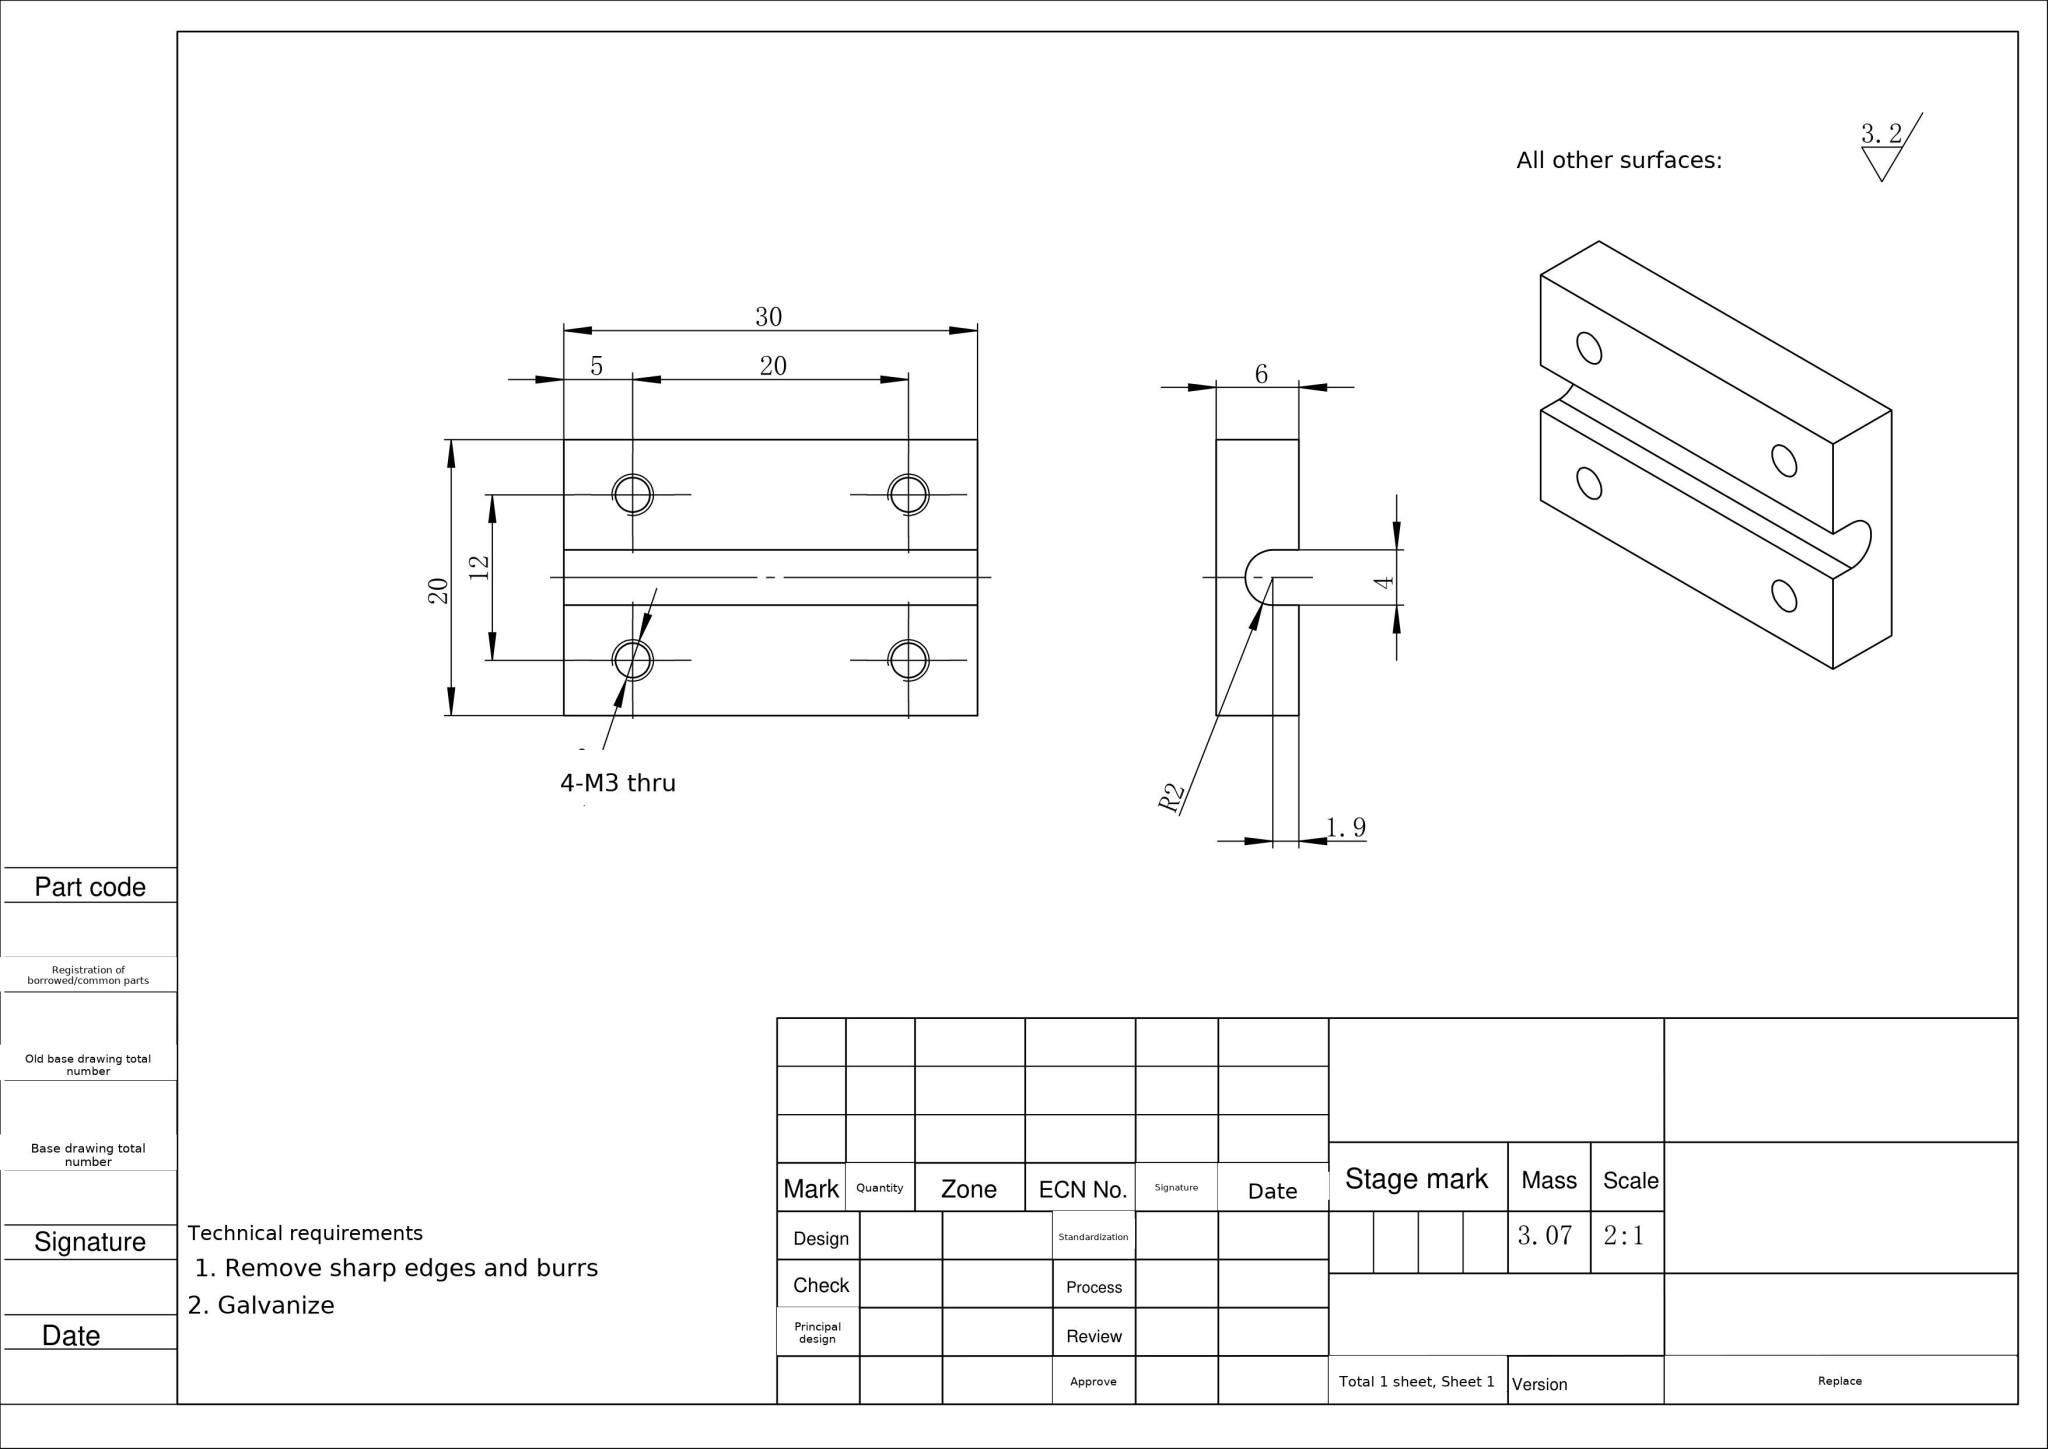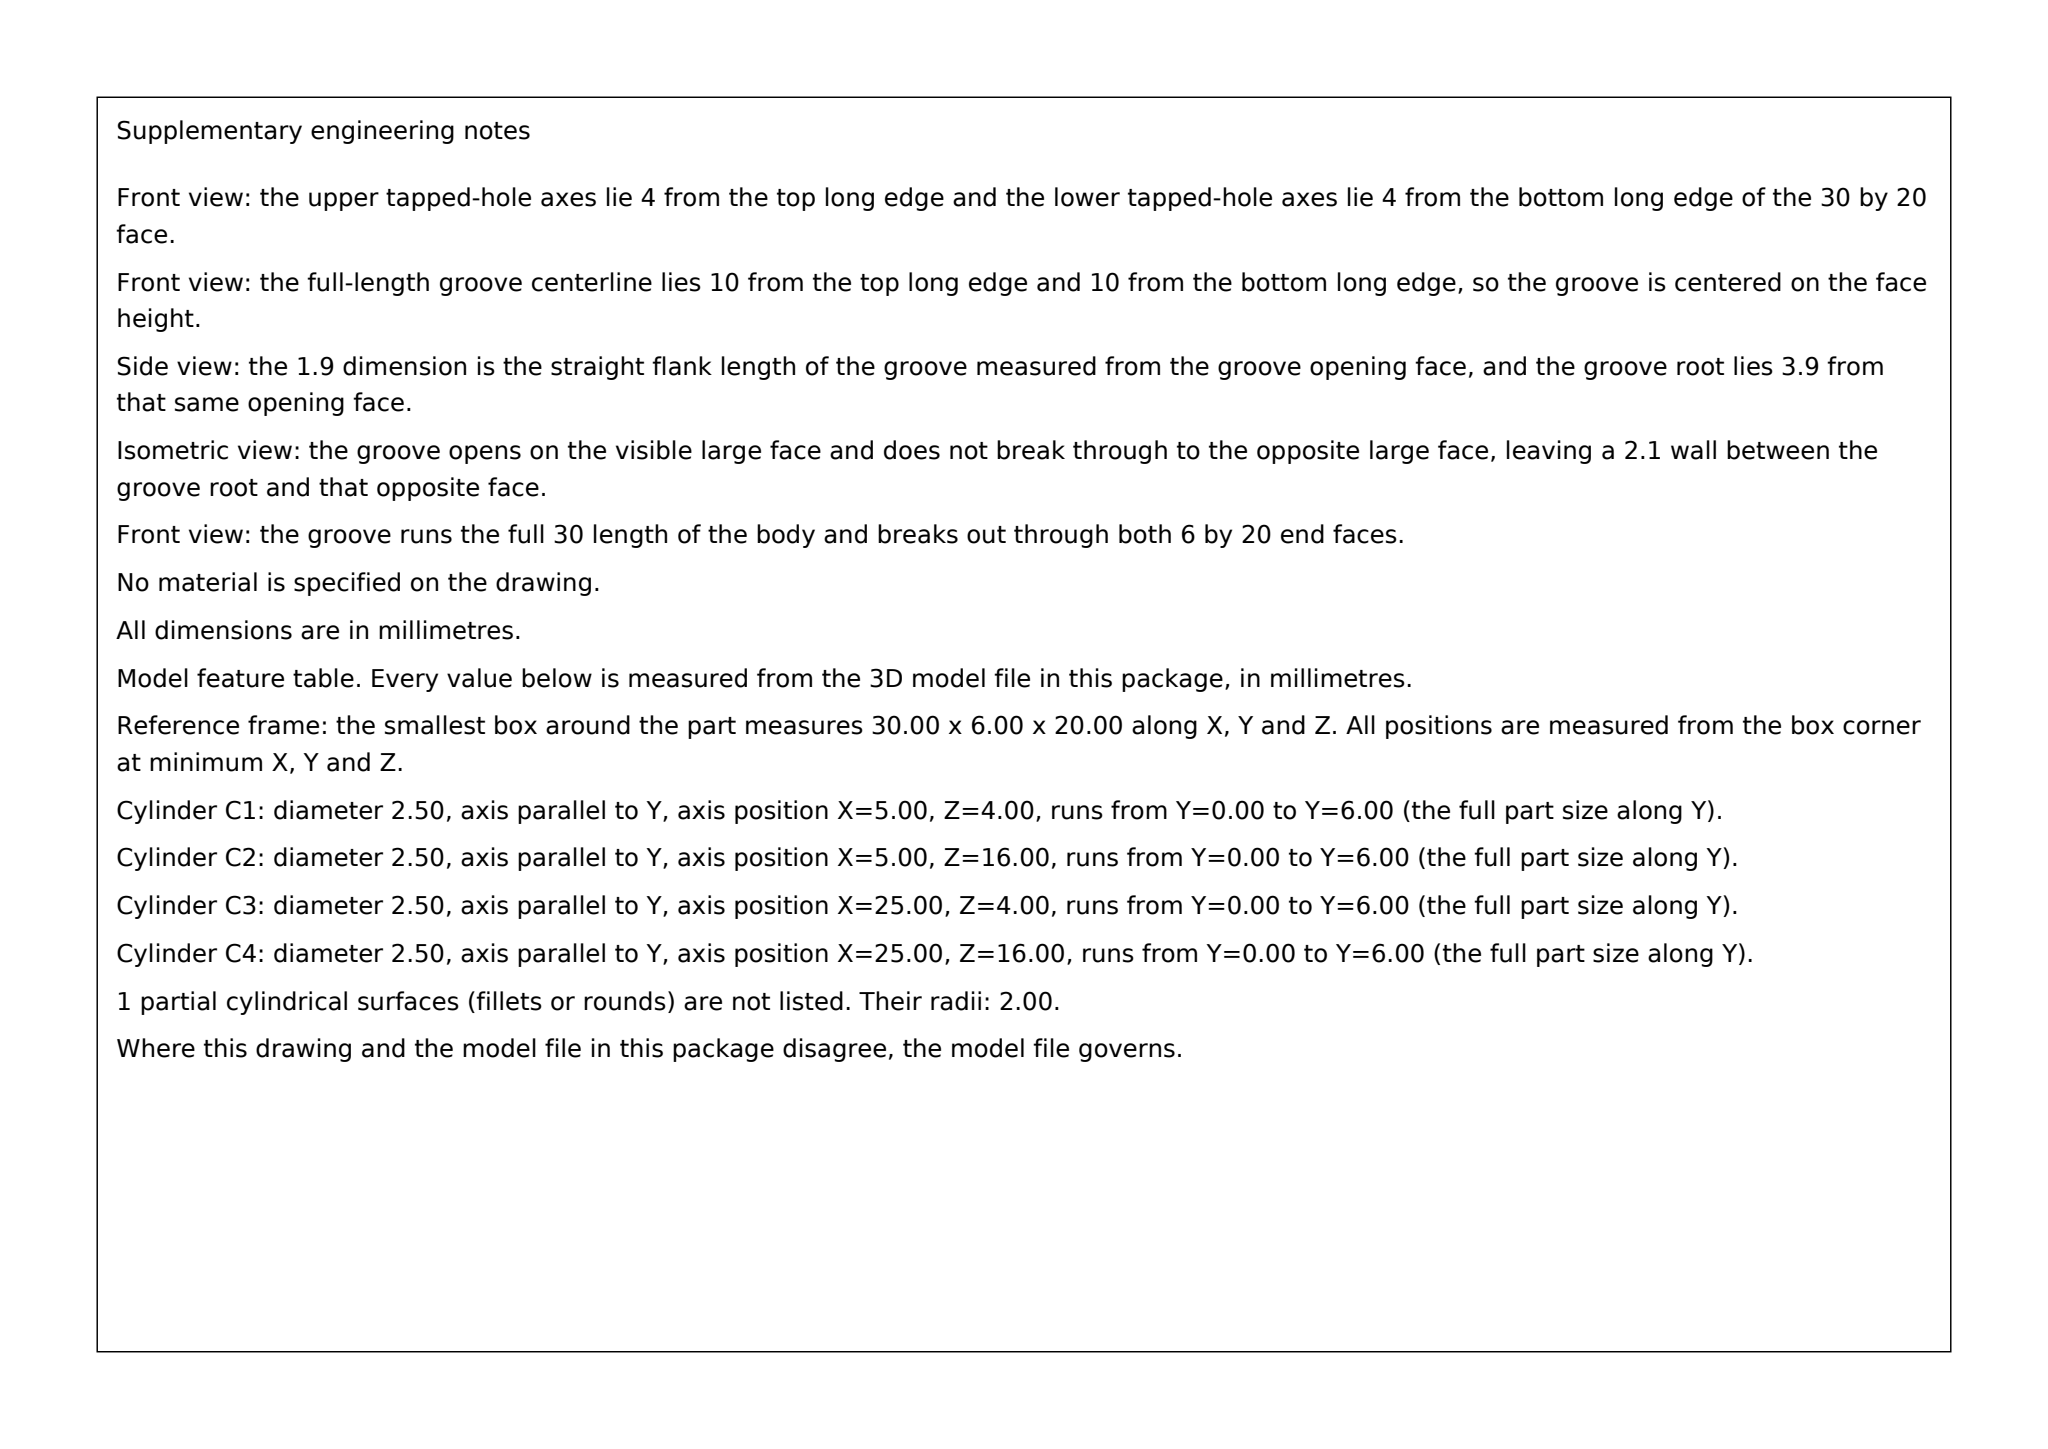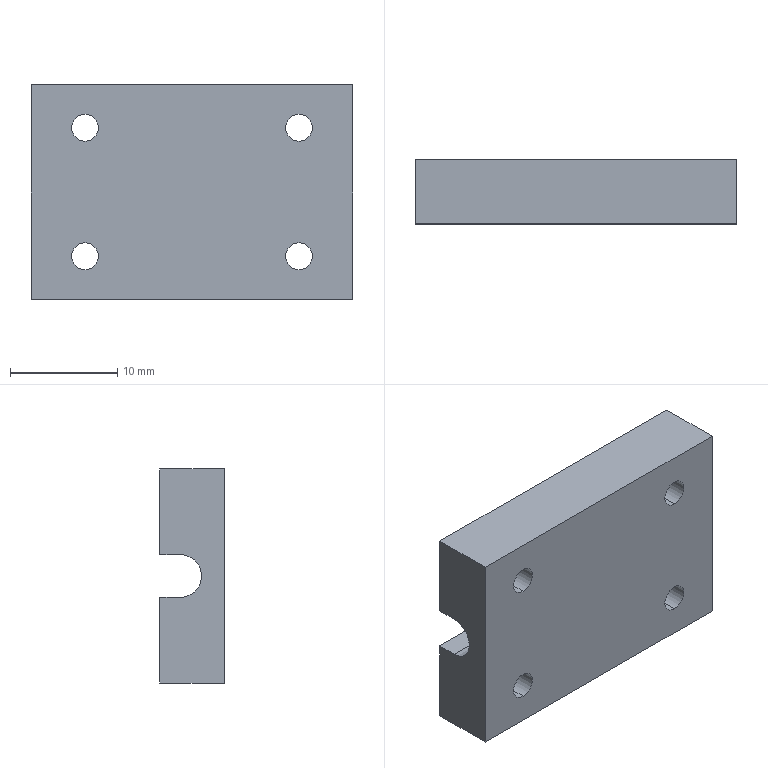Part | SolidWorks | mm | 1 solid | 18 faces | box 30 x 6 x 20 mm | volume 3066 mm3 | cylinder 9 | plane 9 | commonest cylinder face diameters 2.5 x8 4 x1
Drawing notes:
All dimensions in millimetres (mm) unless otherwise stated. | from the solid: STEP model units: mm (bbox_xyz given in mm)
GROOVE: FULL-RADIUS R2 (Ø4) THRU, 30 LONG PARALLEL TO 30 EDGE; AXIS 10 FROM BOTTOM FACE AND 1.9 FROM 6-WIDE FRONT FACE | from the solid: cylinder [4.0,"x",[null,4.1,10.0],30.0] with bbox_xyz [30,6,20] (axis 10 from z=0 face, 4.1 from y=6 face = 1.9 from y=0 face)
build123d program:
from build123d import *

# Parameters (mm, degrees)
SKETCH1_W           = 30
SKETCH1_H           = 20
BOSS_EXTRUDE2_DEPTH = 6
CUT_EXTRUDE1_DEPTH  = 170.118
M3_TAPPED_HOLE1_D   = 2.5


with BuildPart() as part:
    # Sketch1 → Boss-Extrude2 (new body)
    with BuildSketch(Plane(origin=(0, 151, -156), x_dir=(1, 0, 0), z_dir=(0, -1, 0))):
        with Locations((-165.688, 216)):
            Rectangle(SKETCH1_W, SKETCH1_H)
    extrude(amount=BOSS_EXTRUDE2_DEPTH)

    # Sketch2 → Cut-Extrude1 (cut, through all)
    with BuildSketch(Plane.ZY.offset(180.688)):
        with BuildLine():
            Line((58, 149.1), (58, 151))
            Line((58, 151), (62, 151))
            Line((62, 151), (62, 149.1))
            ThreePointArc((62, 149.1), (60, 147.1), (58, 149.1))
        make_face()
    extrude(amount=-CUT_EXTRUDE1_DEPTH, mode=Mode.SUBTRACT)

    # M3 Tapped Hole1 (through all)
    with Locations(Plane(origin=(0, 145, 0), x_dir=(-1, 0, 0), z_dir=(0, -1, 0))):
        with Locations((155.688, -66), (155.688, -54), (175.688, -66), (175.688, -54)):
            Hole(M3_TAPPED_HOLE1_D / 2)


solid = part.part
STEP:
#1=CARTESIAN_POINT('',(-155.688,151.,67.25));
#2=VERTEX_POINT('',#1);
#3=CARTESIAN_POINT('',(-155.688,151.,64.75));
#4=VERTEX_POINT('',#3);
#5=CARTESIAN_POINT('',(-155.688,151.,66.));
#6=DIRECTION('',(0.,-1.,0.));
#7=DIRECTION('',(0.,0.,-1.));
#8=AXIS2_PLACEMENT_3D('',#5,#6,#7);
#9=CIRCLE('',#8,1.25);
#10=EDGE_CURVE('',#2,#4,#9,.T.);
#11=ORIENTED_EDGE('',*,*,#10,.F.);
#12=CARTESIAN_POINT('',(-155.688,145.,67.25));
#13=VERTEX_POINT('',#12);
#14=CARTESIAN_POINT('',(-155.688,145.,67.25));
#15=DIRECTION('',(0.,-1.,0.));
#16=VECTOR('',#15,1000.);
#17=LINE('',#14,#16);
#18=EDGE_CURVE('',#2,#13,#17,.T.);
#19=ORIENTED_EDGE('',*,*,#18,.T.);
#20=CARTESIAN_POINT('',(-155.688,145.,64.75));
#21=VERTEX_POINT('',#20);
#22=CARTESIAN_POINT('',(-155.688,145.,66.));
#23=DIRECTION('',(0.,-1.,0.));
#24=DIRECTION('',(0.,0.,-1.));
#25=AXIS2_PLACEMENT_3D('',#22,#23,#24);
#26=CIRCLE('',#25,1.25);
#27=EDGE_CURVE('',#13,#21,#26,.T.);
#28=ORIENTED_EDGE('',*,*,#27,.T.);
#29=CARTESIAN_POINT('',(-155.688,145.,64.75));
#30=DIRECTION('',(0.,-1.,0.));
#31=VECTOR('',#30,1000.);
#32=LINE('',#29,#31);
#33=EDGE_CURVE('',#4,#21,#32,.T.);
#34=ORIENTED_EDGE('',*,*,#33,.F.);
#35=EDGE_LOOP('',(#11,#19,#28,#34));
#36=FACE_OUTER_BOUND('',#35,.T.);
#37=CARTESIAN_POINT('',(-155.688,145.,66.));
#38=DIRECTION('',(0.,-1.,0.));
#39=DIRECTION('',(0.,0.,-1.));
#40=AXIS2_PLACEMENT_3D('',#37,#38,#39);
#41=CYLINDRICAL_SURFACE('',#40,1.25);
#42=ADVANCED_FACE('',(#36),#41,.F.);
#43=CARTESIAN_POINT('',(-155.688,151.,55.25));
#44=VERTEX_POINT('',#43);
#45=CARTESIAN_POINT('',(-155.688,151.,52.75));
#46=VERTEX_POINT('',#45);
#47=CARTESIAN_POINT('',(-155.688,151.,54.));
#48=DIRECTION('',(0.,-1.,0.));
#49=DIRECTION('',(0.,0.,-1.));
#50=AXIS2_PLACEMENT_3D('',#47,#48,#49);
#51=CIRCLE('',#50,1.25);
#52=EDGE_CURVE('',#44,#46,#51,.T.);
#53=ORIENTED_EDGE('',*,*,#52,.F.);
#54=CARTESIAN_POINT('',(-155.688,145.,55.25));
#55=VERTEX_POINT('',#54);
#56=CARTESIAN_POINT('',(-155.688,145.,55.25));
#57=DIRECTION('',(0.,-1.,0.));
#58=VECTOR('',#57,1000.);
#59=LINE('',#56,#58);
#60=EDGE_CURVE('',#44,#55,#59,.T.);
#61=ORIENTED_EDGE('',*,*,#60,.T.);
#62=CARTESIAN_POINT('',(-155.688,145.,52.75));
#63=VERTEX_POINT('',#62);
#64=CARTESIAN_POINT('',(-155.688,145.,54.));
#65=DIRECTION('',(0.,-1.,0.));
#66=DIRECTION('',(0.,0.,-1.));
#67=AXIS2_PLACEMENT_3D('',#64,#65,#66);
#68=CIRCLE('',#67,1.25);
#69=EDGE_CURVE('',#55,#63,#68,.T.);
#70=ORIENTED_EDGE('',*,*,#69,.T.);
#71=CARTESIAN_POINT('',(-155.688,145.,52.75));
#72=DIRECTION('',(0.,-1.,0.));
#73=VECTOR('',#72,1000.);
#74=LINE('',#71,#73);
#75=EDGE_CURVE('',#46,#63,#74,.T.);
#76=ORIENTED_EDGE('',*,*,#75,.F.);
#77=EDGE_LOOP('',(#53,#61,#70,#76));
#78=FACE_OUTER_BOUND('',#77,.T.);
#79=CARTESIAN_POINT('',(-155.688,145.,54.));
#80=DIRECTION('',(0.,-1.,0.));
#81=DIRECTION('',(0.,0.,-1.));
#82=AXIS2_PLACEMENT_3D('',#79,#80,#81);
#83=CYLINDRICAL_SURFACE('',#82,1.25);
#84=ADVANCED_FACE('',(#78),#83,.F.);
#85=CARTESIAN_POINT('',(-175.688,151.,67.25));
#86=VERTEX_POINT('',#85);
#87=CARTESIAN_POINT('',(-175.688,151.,64.75));
#88=VERTEX_POINT('',#87);
#89=CARTESIAN_POINT('',(-175.688,151.,66.));
#90=DIRECTION('',(0.,-1.,0.));
#91=DIRECTION('',(0.,0.,-1.));
#92=AXIS2_PLACEMENT_3D('',#89,#90,#91);
#93=CIRCLE('',#92,1.25);
#94=EDGE_CURVE('',#86,#88,#93,.T.);
#95=ORIENTED_EDGE('',*,*,#94,.F.);
#96=CARTESIAN_POINT('',(-175.688,145.,67.25));
#97=VERTEX_POINT('',#96);
#98=CARTESIAN_POINT('',(-175.688,145.,67.25));
#99=DIRECTION('',(0.,-1.,0.));
#100=VECTOR('',#99,1000.);
#101=LINE('',#98,#100);
#102=EDGE_CURVE('',#86,#97,#101,.T.);
#103=ORIENTED_EDGE('',*,*,#102,.T.);
#104=CARTESIAN_POINT('',(-175.688,145.,64.75));
#105=VERTEX_POINT('',#104);
#106=CARTESIAN_POINT('',(-175.688,145.,66.));
#107=DIRECTION('',(0.,-1.,0.));
#108=DIRECTION('',(0.,0.,-1.));
#109=AXIS2_PLACEMENT_3D('',#106,#107,#108);
#110=CIRCLE('',#109,1.25);
#111=EDGE_CURVE('',#97,#105,#110,.T.);
#112=ORIENTED_EDGE('',*,*,#111,.T.);
#113=CARTESIAN_POINT('',(-175.688,145.,64.75));
#114=DIRECTION('',(0.,-1.,0.));
#115=VECTOR('',#114,1000.);
#116=LINE('',#113,#115);
#117=EDGE_CURVE('',#88,#105,#116,.T.);
#118=ORIENTED_EDGE('',*,*,#117,.F.);
#119=EDGE_LOOP('',(#95,#103,#112,#118));
#120=FACE_OUTER_BOUND('',#119,.T.);
#121=CARTESIAN_POINT('',(-175.688,145.,66.));
#122=DIRECTION('',(0.,-1.,0.));
#123=DIRECTION('',(0.,0.,-1.));
#124=AXIS2_PLACEMENT_3D('',#121,#122,#123);
#125=CYLINDRICAL_SURFACE('',#124,1.25);
#126=ADVANCED_FACE('',(#120),#125,.F.);
#127=CARTESIAN_POINT('',(-175.688,151.,55.25));
#128=VERTEX_POINT('',#127);
#129=CARTESIAN_POINT('',(-175.688,151.,52.75));
#130=VERTEX_POINT('',#129);
#131=CARTESIAN_POINT('',(-175.688,151.,54.));
#132=DIRECTION('',(0.,-1.,0.));
#133=DIRECTION('',(0.,0.,-1.));
#134=AXIS2_PLACEMENT_3D('',#131,#132,#133);
#135=CIRCLE('',#134,1.25);
#136=EDGE_CURVE('',#128,#130,#135,.T.);
#137=ORIENTED_EDGE('',*,*,#136,.F.);
#138=CARTESIAN_POINT('',(-175.688,145.,55.25));
#139=VERTEX_POINT('',#138);
#140=CARTESIAN_POINT('',(-175.688,145.,55.25));
#141=DIRECTION('',(0.,-1.,0.));
#142=VECTOR('',#141,1000.);
#143=LINE('',#140,#142);
#144=EDGE_CURVE('',#128,#139,#143,.T.);
#145=ORIENTED_EDGE('',*,*,#144,.T.);
#146=CARTESIAN_POINT('',(-175.688,145.,52.75));
#147=VERTEX_POINT('',#146);
#148=CARTESIAN_POINT('',(-175.688,145.,54.));
#149=DIRECTION('',(0.,-1.,0.));
#150=DIRECTION('',(0.,0.,-1.));
#151=AXIS2_PLACEMENT_3D('',#148,#149,#150);
#152=CIRCLE('',#151,1.25);
#153=EDGE_CURVE('',#139,#147,#152,.T.);
#154=ORIENTED_EDGE('',*,*,#153,.T.);
#155=CARTESIAN_POINT('',(-175.688,145.,52.75));
#156=DIRECTION('',(0.,-1.,0.));
#157=VECTOR('',#156,1000.);
#158=LINE('',#155,#157);
#159=EDGE_CURVE('',#130,#147,#158,.T.);
#160=ORIENTED_EDGE('',*,*,#159,.F.);
#161=EDGE_LOOP('',(#137,#145,#154,#160));
#162=FACE_OUTER_BOUND('',#161,.T.);
#163=CARTESIAN_POINT('',(-175.688,145.,54.));
#164=DIRECTION('',(0.,-1.,0.));
#165=DIRECTION('',(0.,0.,-1.));
#166=AXIS2_PLACEMENT_3D('',#163,#164,#165);
#167=CYLINDRICAL_SURFACE('',#166,1.25);
#168=ADVANCED_FACE('',(#162),#167,.F.);
#169=CARTESIAN_POINT('',(-155.688,151.,54.));
#170=DIRECTION('',(0.,-1.,0.));
#171=DIRECTION('',(0.,0.,-1.));
#172=AXIS2_PLACEMENT_3D('',#169,#170,#171);
#173=CIRCLE('',#172,1.25);
#174=EDGE_CURVE('',#46,#44,#173,.T.);
#175=ORIENTED_EDGE('',*,*,#174,.T.);
#176=ORIENTED_EDGE('',*,*,#52,.T.);
#177=EDGE_LOOP('',(#175,#176));
#178=FACE_BOUND('',#177,.T.);
#179=CARTESIAN_POINT('',(-175.688,151.,54.));
#180=DIRECTION('',(0.,-1.,0.));
#181=DIRECTION('',(0.,0.,-1.));
#182=AXIS2_PLACEMENT_3D('',#179,#180,#181);
#183=CIRCLE('',#182,1.25);
#184=EDGE_CURVE('',#130,#128,#183,.T.);
#185=ORIENTED_EDGE('',*,*,#184,.T.);
#186=ORIENTED_EDGE('',*,*,#136,.T.);
#187=EDGE_LOOP('',(#185,#186));
#188=FACE_BOUND('',#187,.T.);
#189=CARTESIAN_POINT('',(-180.688,151.,58.));
#190=VERTEX_POINT('',#189);
#191=CARTESIAN_POINT('',(-180.688,151.,50.));
#192=VERTEX_POINT('',#191);
#193=CARTESIAN_POINT('',(-180.688,151.,70.));
#194=DIRECTION('',(0.,-0.,-1.));
#195=VECTOR('',#194,1000.);
#196=LINE('',#193,#195);
#197=EDGE_CURVE('',#190,#192,#196,.T.);
#198=ORIENTED_EDGE('',*,*,#197,.F.);
#199=CARTESIAN_POINT('',(-150.688,151.,58.));
#200=VERTEX_POINT('',#199);
#201=CARTESIAN_POINT('',(-150.688,151.,58.));
#202=DIRECTION('',(-1.,0.,0.));
#203=VECTOR('',#202,1000.);
#204=LINE('',#201,#203);
#205=EDGE_CURVE('',#200,#190,#204,.T.);
#206=ORIENTED_EDGE('',*,*,#205,.F.);
#207=CARTESIAN_POINT('',(-150.688,151.,50.));
#208=VERTEX_POINT('',#207);
#209=CARTESIAN_POINT('',(-150.688,151.,70.));
#210=DIRECTION('',(0.,0.,1.));
#211=VECTOR('',#210,1000.);
#212=LINE('',#209,#211);
#213=EDGE_CURVE('',#208,#200,#212,.T.);
#214=ORIENTED_EDGE('',*,*,#213,.F.);
#215=CARTESIAN_POINT('',(-180.688,151.,50.));
#216=DIRECTION('',(1.,0.,0.));
#217=VECTOR('',#216,1000.);
#218=LINE('',#215,#217);
#219=EDGE_CURVE('',#192,#208,#218,.T.);
#220=ORIENTED_EDGE('',*,*,#219,.F.);
#221=EDGE_LOOP('',(#198,#206,#214,#220));
#222=FACE_OUTER_BOUND('',#221,.T.);
#223=CARTESIAN_POINT('',(0.,151.,-0.));
#224=DIRECTION('',(0.,-1.,0.));
#225=DIRECTION('',(0.,-0.,-1.));
#226=AXIS2_PLACEMENT_3D('',#223,#224,#225);
#227=PLANE('',#226);
#228=ADVANCED_FACE('',(#178,#188,#222),#227,.F.);
#229=CARTESIAN_POINT('',(-180.688,149.1,58.));
#230=VERTEX_POINT('',#229);
#231=CARTESIAN_POINT('',(-180.688,149.1,62.));
#232=VERTEX_POINT('',#231);
#233=CARTESIAN_POINT('',(-180.688,149.1,60.));
#234=DIRECTION('',(-1.,0.,0.));
#235=DIRECTION('',(0.,0.,1.));
#236=AXIS2_PLACEMENT_3D('',#233,#234,#235);
#237=CIRCLE('',#236,2.);
#238=EDGE_CURVE('',#230,#232,#237,.T.);
#239=ORIENTED_EDGE('',*,*,#238,.F.);
#240=CARTESIAN_POINT('',(-180.688,149.1,58.));
#241=DIRECTION('',(0.,-1.,0.));
#242=VECTOR('',#241,1000.);
#243=LINE('',#240,#242);
#244=EDGE_CURVE('',#190,#230,#243,.T.);
#245=ORIENTED_EDGE('',*,*,#244,.F.);
#246=ORIENTED_EDGE('',*,*,#197,.T.);
#247=CARTESIAN_POINT('',(-180.688,145.,50.));
#248=VERTEX_POINT('',#247);
#249=CARTESIAN_POINT('',(-180.688,145.,50.));
#250=DIRECTION('',(0.,1.,-0.));
#251=VECTOR('',#250,1000.);
#252=LINE('',#249,#251);
#253=EDGE_CURVE('',#248,#192,#252,.T.);
#254=ORIENTED_EDGE('',*,*,#253,.F.);
#255=CARTESIAN_POINT('',(-180.688,145.,70.));
#256=VERTEX_POINT('',#255);
#257=CARTESIAN_POINT('',(-180.688,145.,70.));
#258=DIRECTION('',(0.,-0.,-1.));
#259=VECTOR('',#258,1000.);
#260=LINE('',#257,#259);
#261=EDGE_CURVE('',#256,#248,#260,.T.);
#262=ORIENTED_EDGE('',*,*,#261,.F.);
#263=CARTESIAN_POINT('',(-180.688,151.,70.));
#264=VERTEX_POINT('',#263);
#265=CARTESIAN_POINT('',(-180.688,145.,70.));
#266=DIRECTION('',(0.,1.,-0.));
#267=VECTOR('',#266,1000.);
#268=LINE('',#265,#267);
#269=EDGE_CURVE('',#256,#264,#268,.T.);
#270=ORIENTED_EDGE('',*,*,#269,.T.);
#271=CARTESIAN_POINT('',(-180.688,151.,62.));
#272=VERTEX_POINT('',#271);
#273=CARTESIAN_POINT('',(-180.688,151.,70.));
#274=DIRECTION('',(0.,-0.,-1.));
#275=VECTOR('',#274,1000.);
#276=LINE('',#273,#275);
#277=EDGE_CURVE('',#264,#272,#276,.T.);
#278=ORIENTED_EDGE('',*,*,#277,.T.);
#279=CARTESIAN_POINT('',(-180.688,151.,62.));
#280=DIRECTION('',(0.,1.,0.));
#281=VECTOR('',#280,1000.);
#282=LINE('',#279,#281);
#283=EDGE_CURVE('',#232,#272,#282,.T.);
#284=ORIENTED_EDGE('',*,*,#283,.F.);
#285=EDGE_LOOP('',(#239,#245,#246,#254,#262,#270,#278,#284));
#286=FACE_OUTER_BOUND('',#285,.T.);
#287=CARTESIAN_POINT('',(-180.688,145.,70.));
#288=DIRECTION('',(1.,0.,0.));
#289=DIRECTION('',(0.,0.,-1.));
#290=AXIS2_PLACEMENT_3D('',#287,#288,#289);
#291=PLANE('',#290);
#292=ADVANCED_FACE('',(#286),#291,.F.);
#293=ORIENTED_EDGE('',*,*,#219,.T.);
#294=CARTESIAN_POINT('',(-150.688,145.,50.));
#295=VERTEX_POINT('',#294);
#296=CARTESIAN_POINT('',(-150.688,145.,50.));
#297=DIRECTION('',(0.,1.,-0.));
#298=VECTOR('',#297,1000.);
#299=LINE('',#296,#298);
#300=EDGE_CURVE('',#295,#208,#299,.T.);
#301=ORIENTED_EDGE('',*,*,#300,.F.);
#302=CARTESIAN_POINT('',(-180.688,145.,50.));
#303=DIRECTION('',(1.,0.,0.));
#304=VECTOR('',#303,1000.);
#305=LINE('',#302,#304);
#306=EDGE_CURVE('',#248,#295,#305,.T.);
#307=ORIENTED_EDGE('',*,*,#306,.F.);
#308=ORIENTED_EDGE('',*,*,#253,.T.);
#309=EDGE_LOOP('',(#293,#301,#307,#308));
#310=FACE_OUTER_BOUND('',#309,.T.);
#311=CARTESIAN_POINT('',(-180.688,145.,50.));
#312=DIRECTION('',(0.,0.,1.));
#313=DIRECTION('',(0.,-1.,0.));
#314=AXIS2_PLACEMENT_3D('',#311,#312,#313);
#315=PLANE('',#314);
#316=ADVANCED_FACE('',(#310),#315,.F.);
#317=ORIENTED_EDGE('',*,*,#213,.T.);
#318=CARTESIAN_POINT('',(-150.688,149.1,58.));
#319=VERTEX_POINT('',#318);
#320=CARTESIAN_POINT('',(-150.688,149.1,58.));
#321=DIRECTION('',(0.,-1.,0.));
#322=VECTOR('',#321,1000.);
#323=LINE('',#320,#322);
#324=EDGE_CURVE('',#200,#319,#323,.T.);
#325=ORIENTED_EDGE('',*,*,#324,.T.);
#326=CARTESIAN_POINT('',(-150.688,149.1,62.));
#327=VERTEX_POINT('',#326);
#328=CARTESIAN_POINT('',(-150.688,149.1,60.));
#329=DIRECTION('',(-1.,0.,0.));
#330=DIRECTION('',(0.,0.,1.));
#331=AXIS2_PLACEMENT_3D('',#328,#329,#330);
#332=CIRCLE('',#331,2.);
#333=EDGE_CURVE('',#319,#327,#332,.T.);
#334=ORIENTED_EDGE('',*,*,#333,.T.);
#335=CARTESIAN_POINT('',(-150.688,151.,62.));
#336=VERTEX_POINT('',#335);
#337=CARTESIAN_POINT('',(-150.688,151.,62.));
#338=DIRECTION('',(0.,1.,0.));
#339=VECTOR('',#338,1000.);
#340=LINE('',#337,#339);
#341=EDGE_CURVE('',#327,#336,#340,.T.);
#342=ORIENTED_EDGE('',*,*,#341,.T.);
#343=CARTESIAN_POINT('',(-150.688,151.,70.));
#344=VERTEX_POINT('',#343);
#345=CARTESIAN_POINT('',(-150.688,151.,70.));
#346=DIRECTION('',(0.,0.,1.));
#347=VECTOR('',#346,1000.);
#348=LINE('',#345,#347);
#349=EDGE_CURVE('',#336,#344,#348,.T.);
#350=ORIENTED_EDGE('',*,*,#349,.T.);
#351=CARTESIAN_POINT('',(-150.688,145.,70.));
#352=VERTEX_POINT('',#351);
#353=CARTESIAN_POINT('',(-150.688,145.,70.));
#354=DIRECTION('',(0.,1.,-0.));
#355=VECTOR('',#354,1000.);
#356=LINE('',#353,#355);
#357=EDGE_CURVE('',#352,#344,#356,.T.);
#358=ORIENTED_EDGE('',*,*,#357,.F.);
#359=CARTESIAN_POINT('',(-150.688,145.,70.));
#360=DIRECTION('',(0.,0.,1.));
#361=VECTOR('',#360,1000.);
#362=LINE('',#359,#361);
#363=EDGE_CURVE('',#295,#352,#362,.T.);
#364=ORIENTED_EDGE('',*,*,#363,.F.);
#365=ORIENTED_EDGE('',*,*,#300,.T.);
#366=EDGE_LOOP('',(#317,#325,#334,#342,#350,#358,#364,#365));
#367=FACE_OUTER_BOUND('',#366,.T.);
#368=CARTESIAN_POINT('',(-150.688,145.,70.));
#369=DIRECTION('',(-1.,0.,0.));
#370=DIRECTION('',(0.,0.,1.));
#371=AXIS2_PLACEMENT_3D('',#368,#369,#370);
#372=PLANE('',#371);
#373=ADVANCED_FACE('',(#367),#372,.F.);
#374=CARTESIAN_POINT('',(-180.688,151.,70.));
#375=DIRECTION('',(-1.,0.,0.));
#376=VECTOR('',#375,1000.);
#377=LINE('',#374,#376);
#378=EDGE_CURVE('',#344,#264,#377,.T.);
#379=ORIENTED_EDGE('',*,*,#378,.T.);
#380=ORIENTED_EDGE('',*,*,#269,.F.);
#381=CARTESIAN_POINT('',(-180.688,145.,70.));
#382=DIRECTION('',(-1.,0.,0.));
#383=VECTOR('',#382,1000.);
#384=LINE('',#381,#383);
#385=EDGE_CURVE('',#352,#256,#384,.T.);
#386=ORIENTED_EDGE('',*,*,#385,.F.);
#387=ORIENTED_EDGE('',*,*,#357,.T.);
#388=EDGE_LOOP('',(#379,#380,#386,#387));
#389=FACE_OUTER_BOUND('',#388,.T.);
#390=CARTESIAN_POINT('',(-180.688,145.,70.));
#391=DIRECTION('',(0.,-0.,-1.));
#392=DIRECTION('',(0.,1.,-0.));
#393=AXIS2_PLACEMENT_3D('',#390,#391,#392);
#394=PLANE('',#393);
#395=ADVANCED_FACE('',(#389),#394,.F.);
#396=CARTESIAN_POINT('',(-155.688,145.,66.));
#397=DIRECTION('',(0.,-1.,0.));
#398=DIRECTION('',(0.,0.,-1.));
#399=AXIS2_PLACEMENT_3D('',#396,#397,#398);
#400=CIRCLE('',#399,1.25);
#401=EDGE_CURVE('',#21,#13,#400,.T.);
#402=ORIENTED_EDGE('',*,*,#401,.F.);
#403=ORIENTED_EDGE('',*,*,#27,.F.);
#404=EDGE_LOOP('',(#402,#403));
#405=FACE_BOUND('',#404,.T.);
#406=CARTESIAN_POINT('',(-155.688,145.,54.));
#407=DIRECTION('',(0.,-1.,0.));
#408=DIRECTION('',(0.,0.,-1.));
#409=AXIS2_PLACEMENT_3D('',#406,#407,#408);
#410=CIRCLE('',#409,1.25);
#411=EDGE_CURVE('',#63,#55,#410,.T.);
#412=ORIENTED_EDGE('',*,*,#411,.F.);
#413=ORIENTED_EDGE('',*,*,#69,.F.);
#414=EDGE_LOOP('',(#412,#413));
#415=FACE_BOUND('',#414,.T.);
#416=CARTESIAN_POINT('',(-175.688,145.,66.));
#417=DIRECTION('',(0.,-1.,0.));
#418=DIRECTION('',(0.,0.,-1.));
#419=AXIS2_PLACEMENT_3D('',#416,#417,#418);
#420=CIRCLE('',#419,1.25);
#421=EDGE_CURVE('',#105,#97,#420,.T.);
#422=ORIENTED_EDGE('',*,*,#421,.F.);
#423=ORIENTED_EDGE('',*,*,#111,.F.);
#424=EDGE_LOOP('',(#422,#423));
#425=FACE_BOUND('',#424,.T.);
#426=CARTESIAN_POINT('',(-175.688,145.,54.));
#427=DIRECTION('',(0.,-1.,0.));
#428=DIRECTION('',(0.,0.,-1.));
#429=AXIS2_PLACEMENT_3D('',#426,#427,#428);
#430=CIRCLE('',#429,1.25);
#431=EDGE_CURVE('',#147,#139,#430,.T.);
#432=ORIENTED_EDGE('',*,*,#431,.F.);
#433=ORIENTED_EDGE('',*,*,#153,.F.);
#434=EDGE_LOOP('',(#432,#433));
#435=FACE_BOUND('',#434,.T.);
#436=ORIENTED_EDGE('',*,*,#261,.T.);
#437=ORIENTED_EDGE('',*,*,#306,.T.);
#438=ORIENTED_EDGE('',*,*,#363,.T.);
#439=ORIENTED_EDGE('',*,*,#385,.T.);
#440=EDGE_LOOP('',(#436,#437,#438,#439));
#441=FACE_OUTER_BOUND('',#440,.T.);
#442=CARTESIAN_POINT('',(0.,145.,-0.));
#443=DIRECTION('',(0.,-1.,0.));
#444=DIRECTION('',(0.,-0.,-1.));
#445=AXIS2_PLACEMENT_3D('',#442,#443,#444);
#446=PLANE('',#445);
#447=ADVANCED_FACE('',(#405,#415,#425,#435,#441),#446,.T.);
#448=CARTESIAN_POINT('',(-155.688,151.,66.));
#449=DIRECTION('',(0.,-1.,0.));
#450=DIRECTION('',(0.,0.,-1.));
#451=AXIS2_PLACEMENT_3D('',#448,#449,#450);
#452=CIRCLE('',#451,1.25);
#453=EDGE_CURVE('',#4,#2,#452,.T.);
#454=ORIENTED_EDGE('',*,*,#453,.T.);
#455=ORIENTED_EDGE('',*,*,#10,.T.);
#456=EDGE_LOOP('',(#454,#455));
#457=FACE_BOUND('',#456,.T.);
#458=CARTESIAN_POINT('',(-175.688,151.,66.));
#459=DIRECTION('',(0.,-1.,0.));
#460=DIRECTION('',(0.,0.,-1.));
#461=AXIS2_PLACEMENT_3D('',#458,#459,#460);
#462=CIRCLE('',#461,1.25);
#463=EDGE_CURVE('',#88,#86,#462,.T.);
#464=ORIENTED_EDGE('',*,*,#463,.T.);
#465=ORIENTED_EDGE('',*,*,#94,.T.);
#466=EDGE_LOOP('',(#464,#465));
#467=FACE_BOUND('',#466,.T.);
#468=ORIENTED_EDGE('',*,*,#349,.F.);
#469=CARTESIAN_POINT('',(-150.688,151.,62.));
#470=DIRECTION('',(-1.,0.,0.));
#471=VECTOR('',#470,1000.);
#472=LINE('',#469,#471);
#473=EDGE_CURVE('',#336,#272,#472,.T.);
#474=ORIENTED_EDGE('',*,*,#473,.T.);
#475=ORIENTED_EDGE('',*,*,#277,.F.);
#476=ORIENTED_EDGE('',*,*,#378,.F.);
#477=EDGE_LOOP('',(#468,#474,#475,#476));
#478=FACE_OUTER_BOUND('',#477,.T.);
#479=CARTESIAN_POINT('',(0.,151.,-0.));
#480=DIRECTION('',(0.,-1.,0.));
#481=DIRECTION('',(0.,-0.,-1.));
#482=AXIS2_PLACEMENT_3D('',#479,#480,#481);
#483=PLANE('',#482);
#484=ADVANCED_FACE('',(#457,#467,#478),#483,.F.);
#485=ORIENTED_EDGE('',*,*,#238,.T.);
#486=CARTESIAN_POINT('',(-150.688,149.1,62.));
#487=DIRECTION('',(-1.,0.,0.));
#488=VECTOR('',#487,1000.);
#489=LINE('',#486,#488);
#490=EDGE_CURVE('',#327,#232,#489,.T.);
#491=ORIENTED_EDGE('',*,*,#490,.F.);
#492=ORIENTED_EDGE('',*,*,#333,.F.);
#493=CARTESIAN_POINT('',(-150.688,149.1,58.));
#494=DIRECTION('',(-1.,0.,0.));
#495=VECTOR('',#494,1000.);
#496=LINE('',#493,#495);
#497=EDGE_CURVE('',#319,#230,#496,.T.);
#498=ORIENTED_EDGE('',*,*,#497,.T.);
#499=EDGE_LOOP('',(#485,#491,#492,#498));
#500=FACE_OUTER_BOUND('',#499,.T.);
#501=CARTESIAN_POINT('',(-150.688,149.1,60.));
#502=DIRECTION('',(-1.,0.,0.));
#503=DIRECTION('',(0.,0.,1.));
#504=AXIS2_PLACEMENT_3D('',#501,#502,#503);
#505=CYLINDRICAL_SURFACE('',#504,2.);
#506=ADVANCED_FACE('',(#500),#505,.F.);
#507=ORIENTED_EDGE('',*,*,#244,.T.);
#508=ORIENTED_EDGE('',*,*,#497,.F.);
#509=ORIENTED_EDGE('',*,*,#324,.F.);
#510=ORIENTED_EDGE('',*,*,#205,.T.);
#511=EDGE_LOOP('',(#507,#508,#509,#510));
#512=FACE_OUTER_BOUND('',#511,.T.);
#513=CARTESIAN_POINT('',(-150.688,149.1,58.));
#514=DIRECTION('',(0.,0.,-1.));
#515=DIRECTION('',(-1.,0.,0.));
#516=AXIS2_PLACEMENT_3D('',#513,#514,#515);
#517=PLANE('',#516);
#518=ADVANCED_FACE('',(#512),#517,.F.);
#519=ORIENTED_EDGE('',*,*,#283,.T.);
#520=ORIENTED_EDGE('',*,*,#473,.F.);
#521=ORIENTED_EDGE('',*,*,#341,.F.);
#522=ORIENTED_EDGE('',*,*,#490,.T.);
#523=EDGE_LOOP('',(#519,#520,#521,#522));
#524=FACE_OUTER_BOUND('',#523,.T.);
#525=CARTESIAN_POINT('',(-150.688,151.,62.));
#526=DIRECTION('',(0.,0.,1.));
#527=DIRECTION('',(1.,0.,0.));
#528=AXIS2_PLACEMENT_3D('',#525,#526,#527);
#529=PLANE('',#528);
#530=ADVANCED_FACE('',(#524),#529,.F.);
#531=ORIENTED_EDGE('',*,*,#144,.F.);
#532=ORIENTED_EDGE('',*,*,#184,.F.);
#533=ORIENTED_EDGE('',*,*,#159,.T.);
#534=ORIENTED_EDGE('',*,*,#431,.T.);
#535=EDGE_LOOP('',(#531,#532,#533,#534));
#536=FACE_OUTER_BOUND('',#535,.T.);
#537=CARTESIAN_POINT('',(-175.688,145.,54.));
#538=DIRECTION('',(0.,-1.,0.));
#539=DIRECTION('',(0.,0.,-1.));
#540=AXIS2_PLACEMENT_3D('',#537,#538,#539);
#541=CYLINDRICAL_SURFACE('',#540,1.25);
#542=ADVANCED_FACE('',(#536),#541,.F.);
#543=ORIENTED_EDGE('',*,*,#102,.F.);
#544=ORIENTED_EDGE('',*,*,#463,.F.);
#545=ORIENTED_EDGE('',*,*,#117,.T.);
#546=ORIENTED_EDGE('',*,*,#421,.T.);
#547=EDGE_LOOP('',(#543,#544,#545,#546));
#548=FACE_OUTER_BOUND('',#547,.T.);
#549=CARTESIAN_POINT('',(-175.688,145.,66.));
#550=DIRECTION('',(0.,-1.,0.));
#551=DIRECTION('',(0.,0.,-1.));
#552=AXIS2_PLACEMENT_3D('',#549,#550,#551);
#553=CYLINDRICAL_SURFACE('',#552,1.25);
#554=ADVANCED_FACE('',(#548),#553,.F.);
#555=ORIENTED_EDGE('',*,*,#60,.F.);
#556=ORIENTED_EDGE('',*,*,#174,.F.);
#557=ORIENTED_EDGE('',*,*,#75,.T.);
#558=ORIENTED_EDGE('',*,*,#411,.T.);
#559=EDGE_LOOP('',(#555,#556,#557,#558));
#560=FACE_OUTER_BOUND('',#559,.T.);
#561=CARTESIAN_POINT('',(-155.688,145.,54.));
#562=DIRECTION('',(0.,-1.,0.));
#563=DIRECTION('',(0.,0.,-1.));
#564=AXIS2_PLACEMENT_3D('',#561,#562,#563);
#565=CYLINDRICAL_SURFACE('',#564,1.25);
#566=ADVANCED_FACE('',(#560),#565,.F.);
#567=ORIENTED_EDGE('',*,*,#18,.F.);
#568=ORIENTED_EDGE('',*,*,#453,.F.);
#569=ORIENTED_EDGE('',*,*,#33,.T.);
#570=ORIENTED_EDGE('',*,*,#401,.T.);
#571=EDGE_LOOP('',(#567,#568,#569,#570));
#572=FACE_OUTER_BOUND('',#571,.T.);
#573=CARTESIAN_POINT('',(-155.688,145.,66.));
#574=DIRECTION('',(0.,-1.,0.));
#575=DIRECTION('',(0.,0.,-1.));
#576=AXIS2_PLACEMENT_3D('',#573,#574,#575);
#577=CYLINDRICAL_SURFACE('',#576,1.25);
#578=ADVANCED_FACE('',(#572),#577,.F.);
#579=CLOSED_SHELL('',(#42,#84,#126,#168,#228,#292,#316,#373,#395,#447,#484,#506,#518,#530,#542,#554,#566,#578));
#580=MANIFOLD_SOLID_BREP('',#579);
#581=CARTESIAN_POINT('',(0.,0.,0.));
#582=DIRECTION('',(0.,0.,1.));
#583=DIRECTION('',(1.,0.,0.));
#584=AXIS2_PLACEMENT_3D('',#581,#582,#583);
#585=(LENGTH_UNIT()NAMED_UNIT(*)SI_UNIT(.MILLI.,.METRE.));
#586=UNCERTAINTY_MEASURE_WITH_UNIT(LENGTH_MEASURE(0.00001),#585,'','');
#587=(NAMED_UNIT(*)PLANE_ANGLE_UNIT()SI_UNIT($,.RADIAN.));
#588=(NAMED_UNIT(*)SI_UNIT($,.STERADIAN.)SOLID_ANGLE_UNIT());
#589=(GEOMETRIC_REPRESENTATION_CONTEXT(3)GLOBAL_UNCERTAINTY_ASSIGNED_CONTEXT((#586))GLOBAL_UNIT_ASSIGNED_CONTEXT((#585,#587,#588))REPRESENTATION_CONTEXT('',''));
#590=ADVANCED_BREP_SHAPE_REPRESENTATION('',(#580,#584),#589);